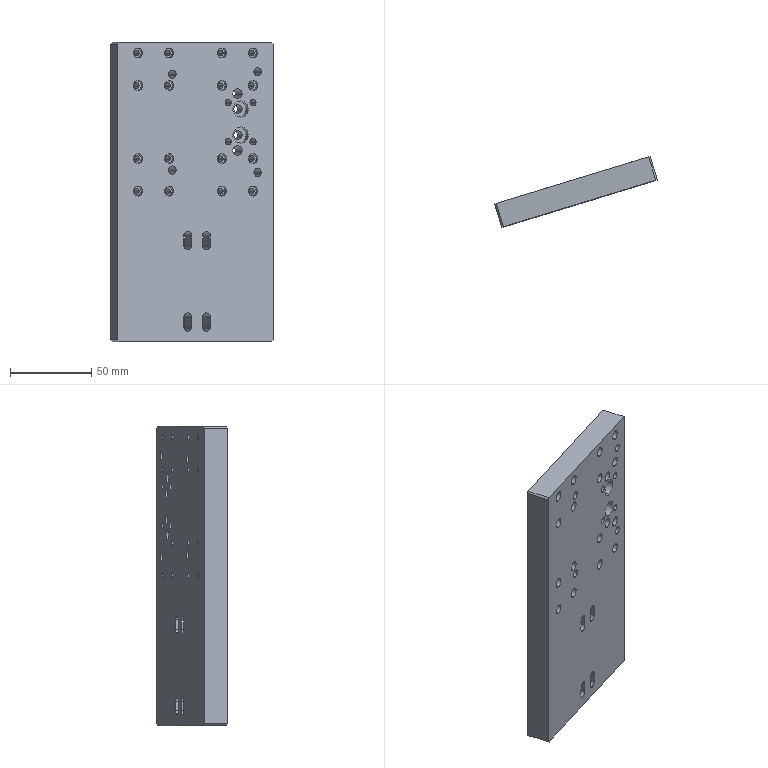Component | SolidWorks | V1ZHXTRotatingSlideRailFixingPlateSB1-1 | 1 solid | 140 faces | box 100.02 x 43.53 x 184 mm | volume 265384 mm3 | cylinder 104 | plane 36 | commonest cylinder face diameters 6 x36 3.5 x32 5.2 x12 5 x8 4 x8 10 x4 5.3 x4
build123d program:
from build123d import *

# Parameters (mm, degrees)
SKETCH1_W                                           = 100
SKETCH1_H                                           = 270
BOSS_EXTRUDE1_DEPTH                                 = 15
CYLINDRICAL_COUNTERSUNK_HOLE_FOR_M3_HEX_D           = 3.5
CYLINDRICAL_COUNTERSUNK_HOLE_FOR_M3_HEX_CBORE_D     = 6
CYLINDRICAL_COUNTERSUNK_HOLE_FOR_M3_HEX_CBORE_DEPTH = 3.5
MIRROR2_COPY_1_D                                    = 3.5
MIRROR2_COPY_1_CBORE_D                              = 6
MIRROR2_COPY_1_CBORE_DEPTH                          = 3.5
SKETCH8_R                                           = 3
CUT_EXTRUDE3_DEPTH                                  = 145.741
M6_TAPPED_HOLE1_D                                   = 5
CUT_EXTRUDE4_DEPTH                                  = 145.741
HOLE_SIZE_FOR_HEX_SOCKET_HEAD_CAP_SCRE_D            = 5.3
HOLE_SIZE_FOR_HEX_SOCKET_HEAD_CAP_SCRE_CBORE_D      = 10
HOLE_SIZE_FOR_HEX_SOCKET_HEAD_CAP_SCRE_CBORE_DEPTH  = 5.7
SKETCH18_R                                          = 2
CUT_EXTRUDE5_DEPTH                                  = 35
SKETCH19_W                                          = 100
SKETCH19_H                                          = 86
CUT_EXTRUDE6_DEPTH                                  = 145.741
M6_TAPPED_HOLE2_D                                   = 5
LPATTERN1_COUNT                                     = 2
LPATTERN1_PITCH                                     = 12
CHAMFER1_SIZE                                       = 1


with BuildPart() as part:
    # Sketch1 → Boss-Extrude1 (new body)
    with BuildSketch(Plane(origin=(0, 0, 0), x_dir=(1, 0, 0), z_dir=(0, 1, 0))):
        Rectangle(SKETCH1_W, SKETCH1_H)
    extrude(amount=BOSS_EXTRUDE1_DEPTH)

    # Cylindrical Countersunk Hole for M3 Hex (through all)
    with Locations(Plane(origin=(0, 15, 0), x_dir=(1, 0, 0), z_dir=(0, 1, 0))):
        with Locations((17, 42.5), (37, 42.5), (37, 22.5), (17, 22.5)):
            cylindrical_countersunk_hole_for_m3_hex = CounterBoreHole(CYLINDRICAL_COUNTERSUNK_HOLE_FOR_M3_HEX_D / 2, CYLINDRICAL_COUNTERSUNK_HOLE_FOR_M3_HEX_CBORE_D / 2, CYLINDRICAL_COUNTERSUNK_HOLE_FOR_M3_HEX_CBORE_DEPTH)

    # Mirror1: Cylindrical Countersunk Hole for M3 Hex across plane
    add(cylindrical_countersunk_hole_for_m3_hex.mirror(Plane.XY), mode=Mode.SUBTRACT)

    # Mirror2: Cylindrical Countersunk Hole for M3 Hex across plane
    add(cylindrical_countersunk_hole_for_m3_hex.mirror(Plane(origin=(0, 0, 0), x_dir=(0, 0, 1), z_dir=(1, 0, 0))), mode=Mode.SUBTRACT)

    # Mirror2 copy 1 (through all)
    with Locations(Plane(origin=(0, 15, 0), x_dir=(-1, 0, 0), z_dir=(0, 1, 0))):
        with Locations((17, 42.5), (37, 42.5), (37, 22.5), (17, 22.5)):
            CounterBoreHole(MIRROR2_COPY_1_D / 2, MIRROR2_COPY_1_CBORE_D / 2, MIRROR2_COPY_1_CBORE_DEPTH)

    # Sketch8 → Cut-Extrude3 (cut, through all)
    with BuildSketch(Plane(origin=(0, 15, 0), x_dir=(1, 0, 0), z_dir=(0, 1, 0))):
        with Locations(Location((27, 17.5, 0), (0, 0, 270))):
            Circle(SKETCH8_R)
        with Locations(Location((27, -17.5, 0), (0, 0, 270))):
            Circle(SKETCH8_R)
    extrude(amount=-CUT_EXTRUDE3_DEPTH, mode=Mode.SUBTRACT)

    # M6 Tapped Hole1 (through all)
    with Locations(Plane(origin=(0, 15, 0), x_dir=(1, 0, 0), z_dir=(0, 1, 0))):
        with Locations((40, 31), (40, -31)):
            Hole(M6_TAPPED_HOLE1_D / 2)

    # Sketch11 → Cut-Extrude4 (cut, through all)
    with BuildSketch(Plane(origin=(0, 15, 0), x_dir=(1, 0, 0), z_dir=(0, 1, 0))):
        with BuildLine():
            Line((9.6, -70), (9.6, -76))
            ThreePointArc((9.6, -76), (7, -78.6), (4.4, -76))
            Line((4.4, -76), (4.4, -70))
            ThreePointArc((4.4, -70), (7, -67.4), (9.6, -70))
        make_face()
        with BuildLine():
            Line((9.6, -120), (9.6, -126))
            ThreePointArc((9.6, -126), (7, -128.6), (4.4, -126))
            Line((4.4, -126), (4.4, -120))
            ThreePointArc((4.4, -120), (7, -117.4), (9.6, -120))
        make_face()
    cut_extrude4 = extrude(amount=-CUT_EXTRUDE4_DEPTH, mode=Mode.SUBTRACT)

    # Hole Size _for_ Hex Socket Head Cap Scre (through all)
    with Locations(Plane(origin=(0, 15, 0), x_dir=(1, 0, 0), z_dir=(0, 1, 0))):
        with Locations((29, 8), (29, -8)):
            CounterBoreHole(HOLE_SIZE_FOR_HEX_SOCKET_HEAD_CAP_SCRE_D / 2, HOLE_SIZE_FOR_HEX_SOCKET_HEAD_CAP_SCRE_CBORE_D / 2, HOLE_SIZE_FOR_HEX_SOCKET_HEAD_CAP_SCRE_CBORE_DEPTH)

    # Sketch18 → Cut-Extrude5 (cut)
    with BuildSketch(Plane(origin=(0, 15, 0), x_dir=(1, 0, 0), z_dir=(0, 1, 0))):
        with Locations(Location((21, 12, 0), (0, 0, 270))):
            Circle(SKETCH18_R)
        with Locations(Location((37, 12, 0), (0, 0, 270))):
            Circle(SKETCH18_R)
        with Locations(Location((37, -12, 0), (0, 0, 90))):
            Circle(SKETCH18_R)
        with Locations(Location((21, -12, 0), (0, 0, 90))):
            Circle(SKETCH18_R)
    extrude(amount=-CUT_EXTRUDE5_DEPTH, mode=Mode.SUBTRACT)

    # Sketch19 → Cut-Extrude6 (cut, through all)
    with BuildSketch(Plane.XZ):
        with Locations((0, -92)):
            Rectangle(SKETCH19_W, SKETCH19_H)
    extrude(amount=-CUT_EXTRUDE6_DEPTH, mode=Mode.SUBTRACT)

    # M6 Tapped Hole2 (through all)
    with Locations(Plane(origin=(0, 15, 0), x_dir=(1, 0, 0), z_dir=(0, 1, 0))):
        with Locations((-15, 29.5), (-15, -29.5)):
            Hole(M6_TAPPED_HOLE2_D / 2)

    # LPattern1: Cut-Extrude4 ×2
    with Locations(*[(-i * LPATTERN1_PITCH, 0, 0) for i in range(1, LPATTERN1_COUNT)]):
        add(cut_extrude4, mode=Mode.SUBTRACT)

    # Chamfer1
    chamfer1_edges = [part.edges().sort_by_distance(p)[0] for p in [
        (50, 7.5, -49),
        (-50, 7.5, -49),
        (50, 7.5, 135),
        (-50, 7.5, 135),
    ]]
    chamfer(chamfer1_edges, length=CHAMFER1_SIZE)


solid = part.part

# Placed as in the assembly
solid = solid.moved(Location((163.536, -178.819, 375.239), (-180, 0, -16.968)))